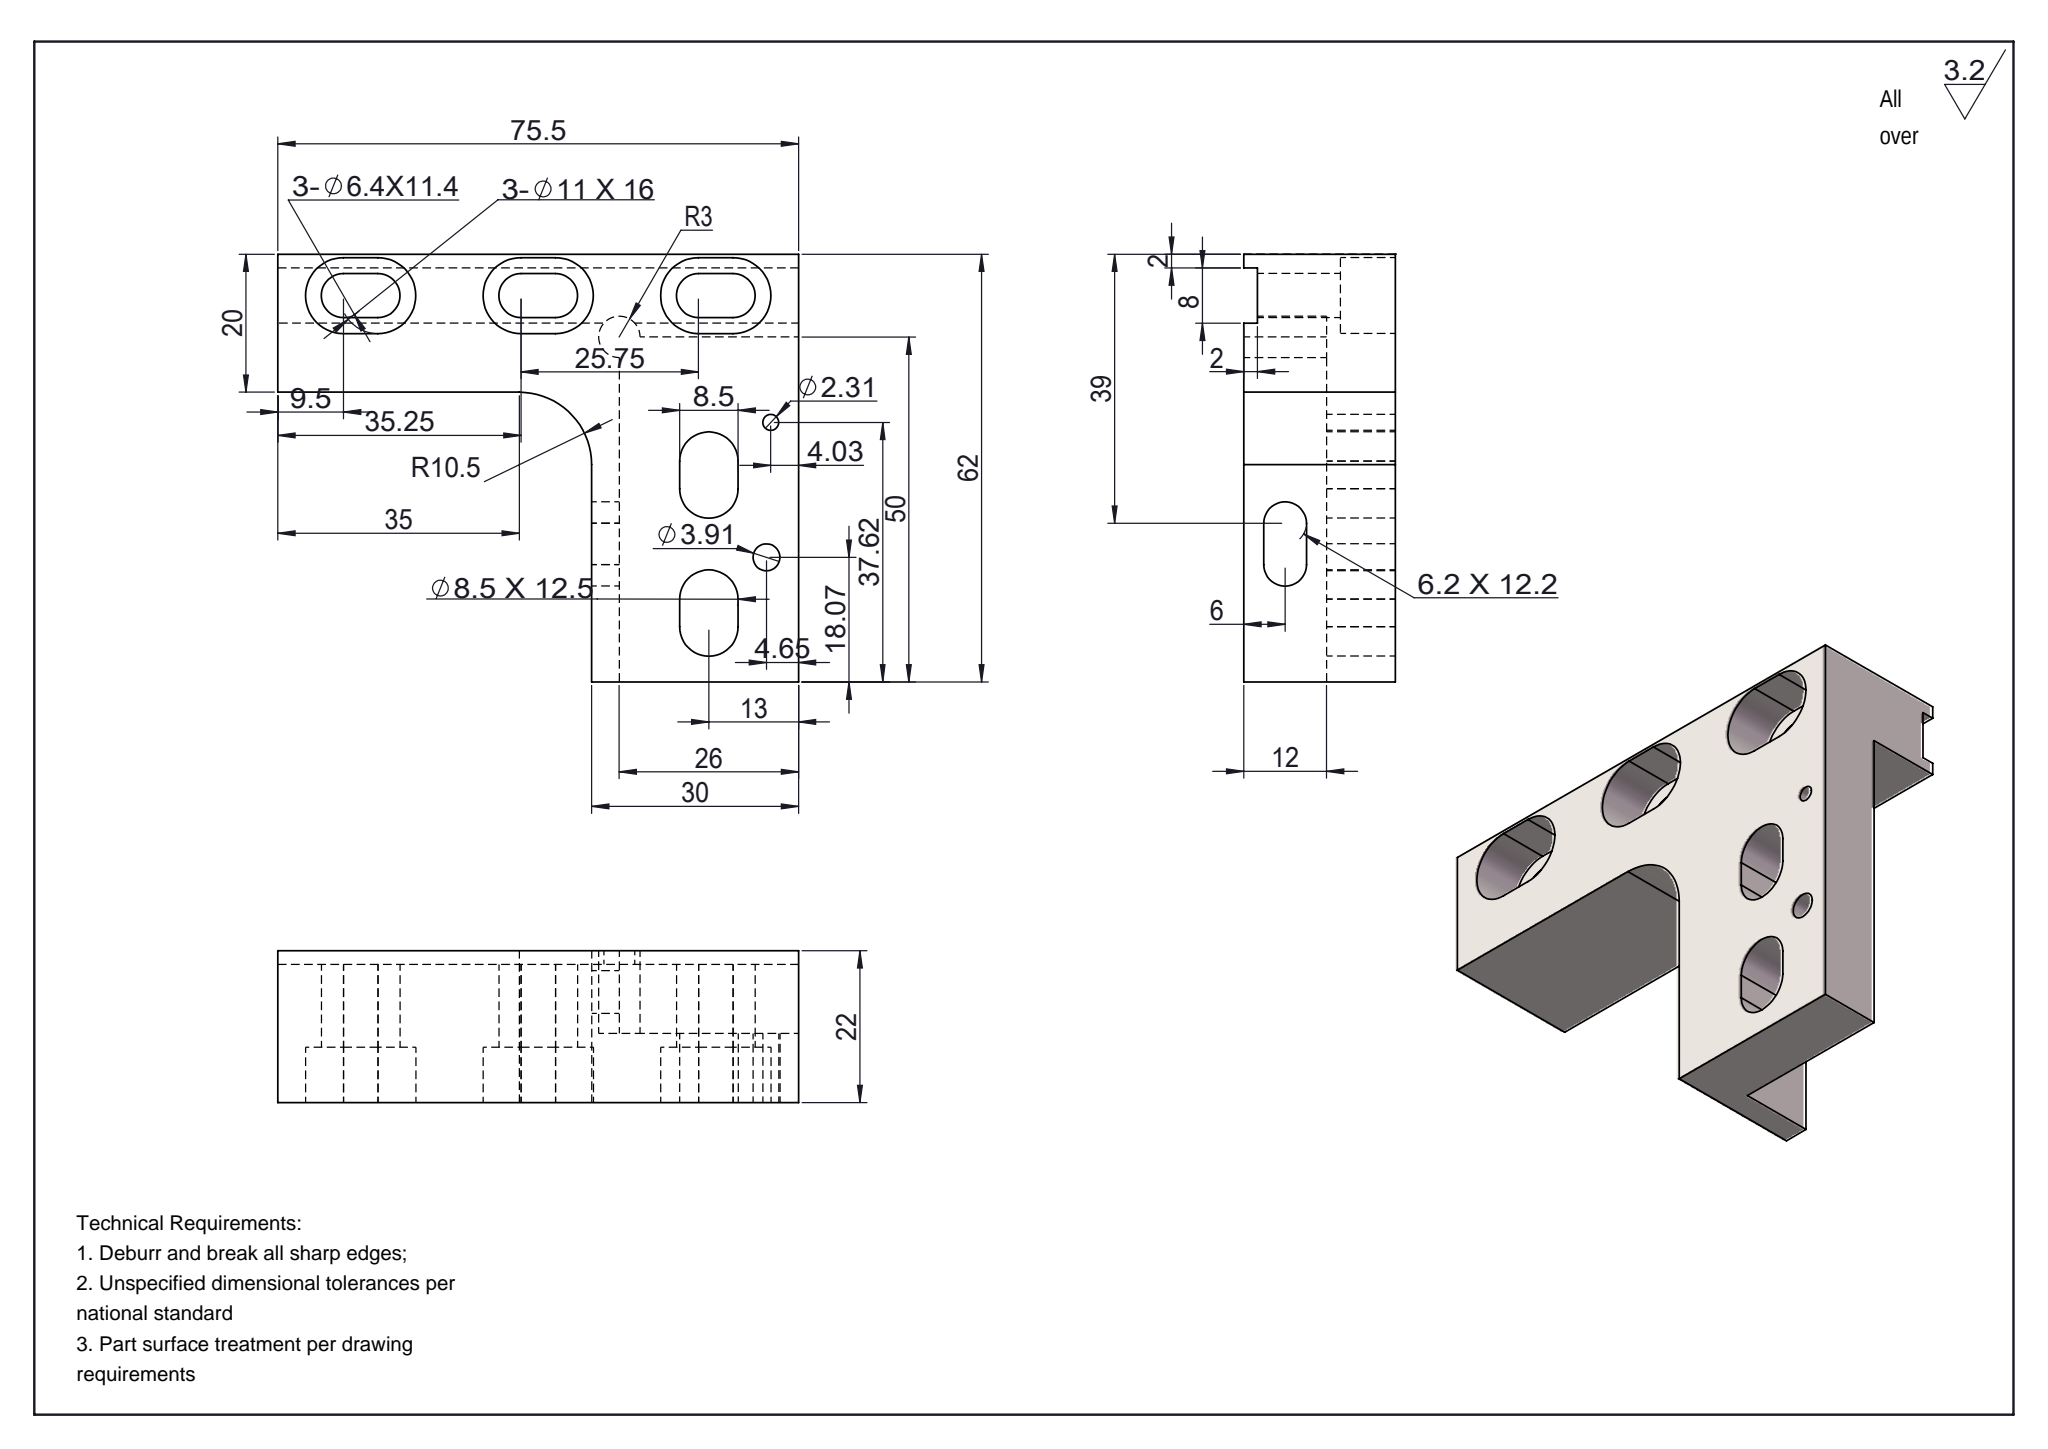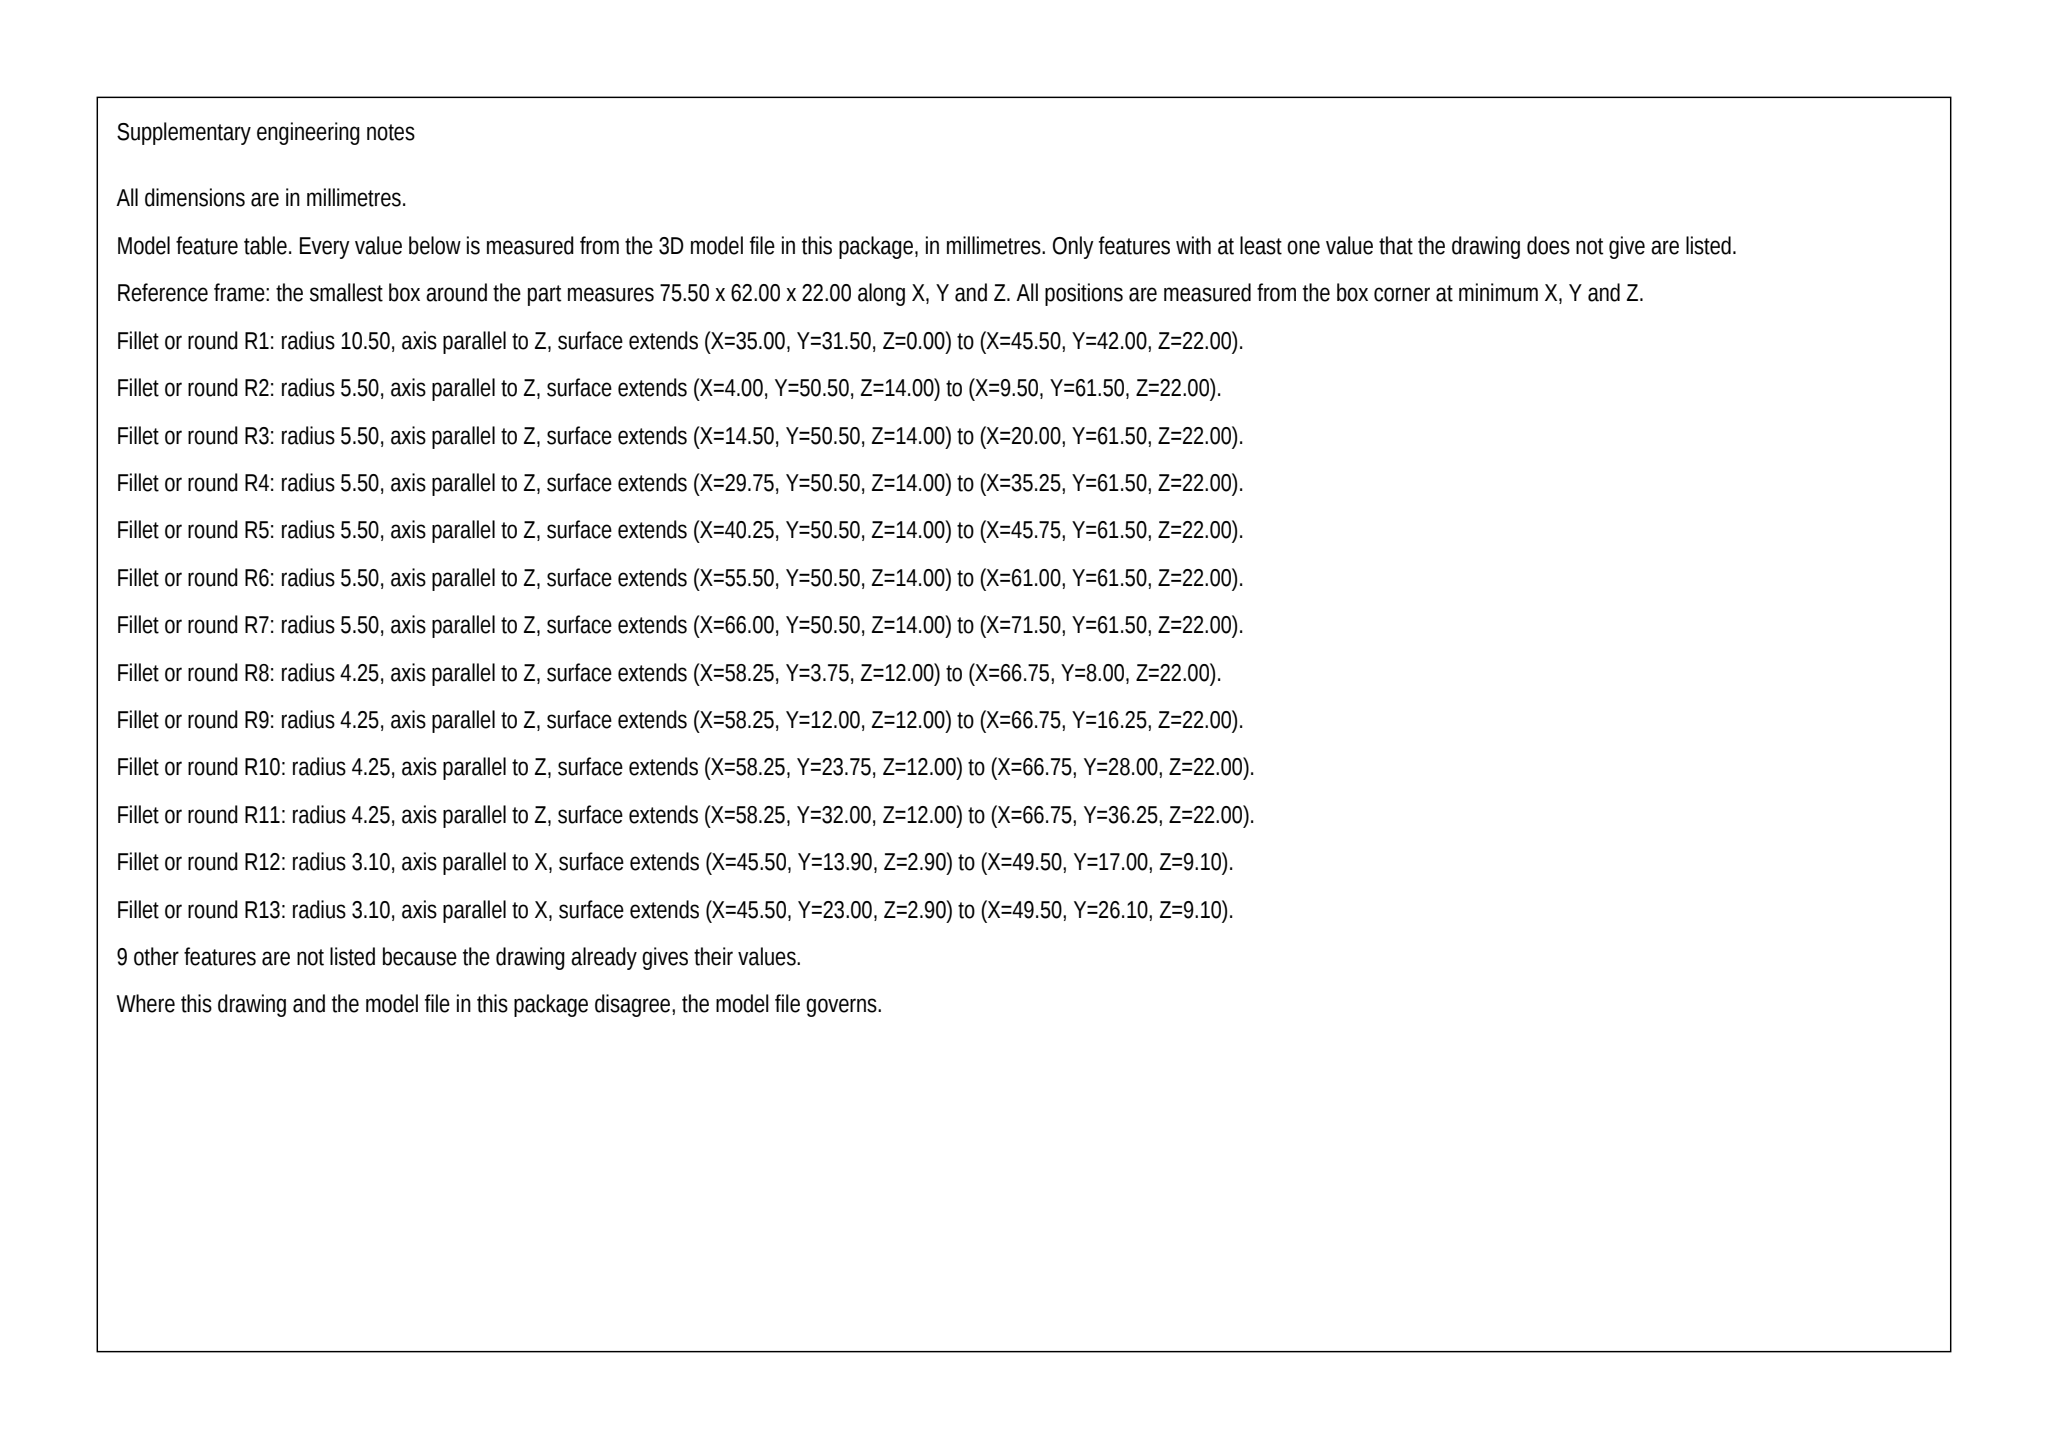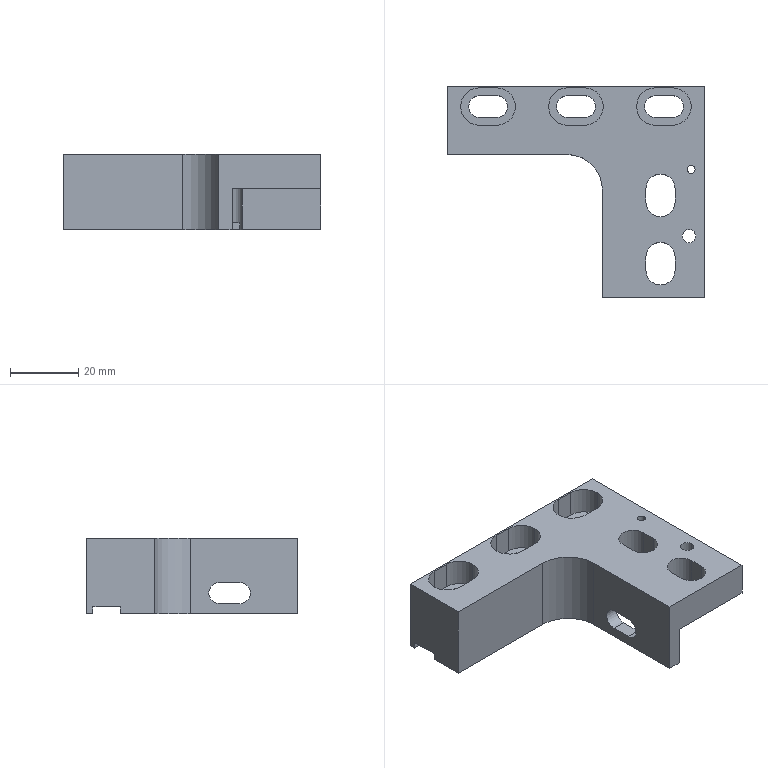Part | SolidWorks | mm | 1 solid | 69 faces | box 75.5 x 62 x 22 mm | volume 36245 mm3 | plane 38 | cylinder 31 | commonest cylinder face diameters 6.4 x9 11 x9 8.5 x4 3.911 x2 2.311 x2 6 x2 6.2 x2 20.994 x1